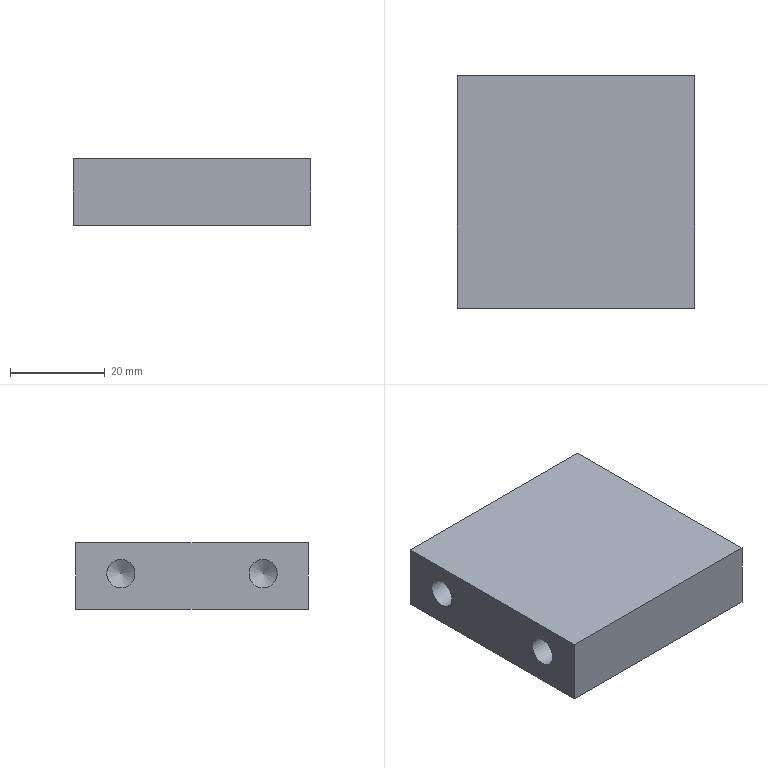Component | NX | BASE_PLATE | 1 solid | 16 faces | box 50 x 49 x 14 mm | volume 32394 mm3 | plane 6 | cone 5 | cylinder 5 | commonest cylinder face diameters 6 x4 4 x1
STEP:
#1=CARTESIAN_POINT('',(0.,0.,0.));
#2=DIRECTION('',(0.,0.,1.));
#3=DIRECTION('',(1.,0.,0.));
#4=AXIS2_PLACEMENT_3D('',#1,#2,#3);
#5=CARTESIAN_POINT('',(25.,0.,2.5));
#6=VERTEX_POINT('',#5);
#7=CARTESIAN_POINT('',(25.,0.,0.5));
#8=DIRECTION('',(-1.,0.,0.));
#9=DIRECTION('',(0.,0.,1.));
#10=AXIS2_PLACEMENT_3D('',#7,#8,#9);
#11=CIRCLE('',#10,2.);
#12=CARTESIAN_POINT('',(25.,-24.5,7.));
#13=DIRECTION('',(-1.,0.,0.));
#14=DIRECTION('',(0.,0.,1.));
#15=AXIS2_PLACEMENT_3D('',#12,#13,#14);
#16=PLANE('',#15);
#17=CARTESIAN_POINT('',(-6.5,24.5));
#18=DIRECTION('',(1.,0.));
#19=AXIS2_PLACEMENT_2D('',#17,#18);
#20=CIRCLE('',#19,2.);
#21=(GEOMETRIC_REPRESENTATION_CONTEXT(2)PARAMETRIC_REPRESENTATION_CONTEXT()REPRESENTATION_CONTEXT('',''));
#22=DEFINITIONAL_REPRESENTATION('',(#20),#21);
#23=PCURVE('',#16,#22);
#24=CARTESIAN_POINT('',(25.,0.,0.5));
#25=DIRECTION('',(-1.,0.,0.));
#26=DIRECTION('',(0.,0.,1.));
#27=AXIS2_PLACEMENT_3D('',#24,#25,#26);
#28=CYLINDRICAL_SURFACE('',#27,2.);
#29=CARTESIAN_POINT('',(0.,0.));
#30=DIRECTION('',(1.,0.));
#31=VECTOR('',#30,1.);
#32=LINE('',#29,#31);
#33=(GEOMETRIC_REPRESENTATION_CONTEXT(2)PARAMETRIC_REPRESENTATION_CONTEXT()REPRESENTATION_CONTEXT('',''));
#34=DEFINITIONAL_REPRESENTATION('',(#32),#33);
#35=PCURVE('',#28,#34);
#36=SURFACE_CURVE('',#11,(#23,#35),.PCURVE_S1.);
#37=EDGE_CURVE('',#6,#6,#36,.T.);
#38=ORIENTED_EDGE('',*,*,#37,.T.);
#39=EDGE_LOOP('',(#38));
#40=FACE_BOUND('',#39,.T.);
#41=CARTESIAN_POINT('',(25.,15.,3.5));
#42=VERTEX_POINT('',#41);
#43=CARTESIAN_POINT('',(25.,15.,0.5));
#44=DIRECTION('',(-1.,0.,0.));
#45=DIRECTION('',(0.,0.,1.));
#46=AXIS2_PLACEMENT_3D('',#43,#44,#45);
#47=CIRCLE('',#46,3.);
#48=CARTESIAN_POINT('',(-6.5,39.5));
#49=DIRECTION('',(1.,0.));
#50=AXIS2_PLACEMENT_2D('',#48,#49);
#51=CIRCLE('',#50,3.);
#52=(GEOMETRIC_REPRESENTATION_CONTEXT(2)PARAMETRIC_REPRESENTATION_CONTEXT()REPRESENTATION_CONTEXT('',''));
#53=DEFINITIONAL_REPRESENTATION('',(#51),#52);
#54=PCURVE('',#16,#53);
#55=CARTESIAN_POINT('',(25.,15.,0.5));
#56=DIRECTION('',(-1.,0.,0.));
#57=DIRECTION('',(0.,0.,1.));
#58=AXIS2_PLACEMENT_3D('',#55,#56,#57);
#59=CYLINDRICAL_SURFACE('',#58,3.);
#60=CARTESIAN_POINT('',(0.,0.));
#61=DIRECTION('',(1.,0.));
#62=VECTOR('',#61,1.);
#63=LINE('',#60,#62);
#64=(GEOMETRIC_REPRESENTATION_CONTEXT(2)PARAMETRIC_REPRESENTATION_CONTEXT()REPRESENTATION_CONTEXT('',''));
#65=DEFINITIONAL_REPRESENTATION('',(#63),#64);
#66=PCURVE('',#59,#65);
#67=SURFACE_CURVE('',#47,(#54,#66),.PCURVE_S1.);
#68=EDGE_CURVE('',#42,#42,#67,.T.);
#69=ORIENTED_EDGE('',*,*,#68,.T.);
#70=EDGE_LOOP('',(#69));
#71=FACE_BOUND('',#70,.T.);
#72=CARTESIAN_POINT('',(25.,-15.,3.5));
#73=VERTEX_POINT('',#72);
#74=CARTESIAN_POINT('',(25.,-15.,0.5));
#75=DIRECTION('',(-1.,0.,0.));
#76=DIRECTION('',(0.,0.,1.));
#77=AXIS2_PLACEMENT_3D('',#74,#75,#76);
#78=CIRCLE('',#77,3.);
#79=CARTESIAN_POINT('',(-6.5,9.5));
#80=DIRECTION('',(1.,0.));
#81=AXIS2_PLACEMENT_2D('',#79,#80);
#82=CIRCLE('',#81,3.);
#83=(GEOMETRIC_REPRESENTATION_CONTEXT(2)PARAMETRIC_REPRESENTATION_CONTEXT()REPRESENTATION_CONTEXT('',''));
#84=DEFINITIONAL_REPRESENTATION('',(#82),#83);
#85=PCURVE('',#16,#84);
#86=CARTESIAN_POINT('',(25.,-15.,0.5));
#87=DIRECTION('',(-1.,0.,0.));
#88=DIRECTION('',(0.,0.,1.));
#89=AXIS2_PLACEMENT_3D('',#86,#87,#88);
#90=CYLINDRICAL_SURFACE('',#89,3.);
#91=CARTESIAN_POINT('',(0.,0.));
#92=DIRECTION('',(1.,0.));
#93=VECTOR('',#92,1.);
#94=LINE('',#91,#93);
#95=(GEOMETRIC_REPRESENTATION_CONTEXT(2)PARAMETRIC_REPRESENTATION_CONTEXT()REPRESENTATION_CONTEXT('',''));
#96=DEFINITIONAL_REPRESENTATION('',(#94),#95);
#97=PCURVE('',#90,#96);
#98=SURFACE_CURVE('',#78,(#85,#97),.PCURVE_S1.);
#99=EDGE_CURVE('',#73,#73,#98,.T.);
#100=ORIENTED_EDGE('',*,*,#99,.T.);
#101=EDGE_LOOP('',(#100));
#102=FACE_BOUND('',#101,.T.);
#103=CARTESIAN_POINT('',(25.,-24.5,-7.));
#104=VERTEX_POINT('',#103);
#105=CARTESIAN_POINT('',(25.,24.5,-7.));
#106=VERTEX_POINT('',#105);
#107=CARTESIAN_POINT('',(25.,-24.5,-7.));
#108=DIRECTION('',(0.,1.,0.));
#109=VECTOR('',#108,1.);
#110=LINE('',#107,#109);
#111=CARTESIAN_POINT('',(-14.,0.));
#112=DIRECTION('',(0.,1.));
#113=VECTOR('',#112,1.);
#114=LINE('',#111,#113);
#115=(GEOMETRIC_REPRESENTATION_CONTEXT(2)PARAMETRIC_REPRESENTATION_CONTEXT()REPRESENTATION_CONTEXT('',''));
#116=DEFINITIONAL_REPRESENTATION('',(#114),#115);
#117=PCURVE('',#16,#116);
#118=CARTESIAN_POINT('',(-25.,-24.5,-7.));
#119=DIRECTION('',(0.,0.,1.));
#120=DIRECTION('',(1.,0.,0.));
#121=AXIS2_PLACEMENT_3D('',#118,#119,#120);
#122=PLANE('',#121);
#123=CARTESIAN_POINT('',(50.,0.));
#124=DIRECTION('',(0.,1.));
#125=VECTOR('',#124,1.);
#126=LINE('',#123,#125);
#127=(GEOMETRIC_REPRESENTATION_CONTEXT(2)PARAMETRIC_REPRESENTATION_CONTEXT()REPRESENTATION_CONTEXT('',''));
#128=DEFINITIONAL_REPRESENTATION('',(#126),#127);
#129=PCURVE('',#122,#128);
#130=SURFACE_CURVE('',#110,(#117,#129),.PCURVE_S1.);
#131=EDGE_CURVE('',#104,#106,#130,.T.);
#132=ORIENTED_EDGE('',*,*,#131,.T.);
#133=CARTESIAN_POINT('',(25.,24.5,7.));
#134=VERTEX_POINT('',#133);
#135=CARTESIAN_POINT('',(25.,24.5,7.));
#136=DIRECTION('',(0.,0.,-1.));
#137=VECTOR('',#136,1.);
#138=LINE('',#135,#137);
#139=CARTESIAN_POINT('',(0.,49.));
#140=DIRECTION('',(-1.,0.));
#141=VECTOR('',#140,1.);
#142=LINE('',#139,#141);
#143=(GEOMETRIC_REPRESENTATION_CONTEXT(2)PARAMETRIC_REPRESENTATION_CONTEXT()REPRESENTATION_CONTEXT('',''));
#144=DEFINITIONAL_REPRESENTATION('',(#142),#143);
#145=PCURVE('',#16,#144);
#146=CARTESIAN_POINT('',(25.,24.5,7.));
#147=DIRECTION('',(0.,-1.,0.));
#148=DIRECTION('',(1.,0.,0.));
#149=AXIS2_PLACEMENT_3D('',#146,#147,#148);
#150=PLANE('',#149);
#151=CARTESIAN_POINT('',(0.,0.));
#152=DIRECTION('',(0.,-1.));
#153=VECTOR('',#152,1.);
#154=LINE('',#151,#153);
#155=(GEOMETRIC_REPRESENTATION_CONTEXT(2)PARAMETRIC_REPRESENTATION_CONTEXT()REPRESENTATION_CONTEXT('',''));
#156=DEFINITIONAL_REPRESENTATION('',(#154),#155);
#157=PCURVE('',#150,#156);
#158=SURFACE_CURVE('',#138,(#145,#157),.PCURVE_S1.);
#159=EDGE_CURVE('',#134,#106,#158,.T.);
#160=ORIENTED_EDGE('',*,*,#159,.F.);
#161=CARTESIAN_POINT('',(25.,-24.5,7.));
#162=VERTEX_POINT('',#161);
#163=CARTESIAN_POINT('',(25.,-24.5,7.));
#164=DIRECTION('',(0.,1.,0.));
#165=VECTOR('',#164,1.);
#166=LINE('',#163,#165);
#167=CARTESIAN_POINT('',(0.,0.));
#168=DIRECTION('',(0.,1.));
#169=VECTOR('',#168,1.);
#170=LINE('',#167,#169);
#171=(GEOMETRIC_REPRESENTATION_CONTEXT(2)PARAMETRIC_REPRESENTATION_CONTEXT()REPRESENTATION_CONTEXT('',''));
#172=DEFINITIONAL_REPRESENTATION('',(#170),#171);
#173=PCURVE('',#16,#172);
#174=CARTESIAN_POINT('',(-25.,-24.5,7.));
#175=DIRECTION('',(0.,0.,1.));
#176=DIRECTION('',(1.,0.,0.));
#177=AXIS2_PLACEMENT_3D('',#174,#175,#176);
#178=PLANE('',#177);
#179=CARTESIAN_POINT('',(50.,0.));
#180=DIRECTION('',(0.,1.));
#181=VECTOR('',#180,1.);
#182=LINE('',#179,#181);
#183=(GEOMETRIC_REPRESENTATION_CONTEXT(2)PARAMETRIC_REPRESENTATION_CONTEXT()REPRESENTATION_CONTEXT('',''));
#184=DEFINITIONAL_REPRESENTATION('',(#182),#183);
#185=PCURVE('',#178,#184);
#186=SURFACE_CURVE('',#166,(#173,#185),.PCURVE_S1.);
#187=EDGE_CURVE('',#162,#134,#186,.T.);
#188=ORIENTED_EDGE('',*,*,#187,.F.);
#189=CARTESIAN_POINT('',(25.,-24.5,7.));
#190=DIRECTION('',(0.,0.,-1.));
#191=VECTOR('',#190,1.);
#192=LINE('',#189,#191);
#193=CARTESIAN_POINT('',(0.,0.));
#194=DIRECTION('',(-1.,0.));
#195=VECTOR('',#194,1.);
#196=LINE('',#193,#195);
#197=(GEOMETRIC_REPRESENTATION_CONTEXT(2)PARAMETRIC_REPRESENTATION_CONTEXT()REPRESENTATION_CONTEXT('',''));
#198=DEFINITIONAL_REPRESENTATION('',(#196),#197);
#199=PCURVE('',#16,#198);
#200=CARTESIAN_POINT('',(-25.,-24.5,7.));
#201=DIRECTION('',(0.,1.,0.));
#202=DIRECTION('',(0.,0.,1.));
#203=AXIS2_PLACEMENT_3D('',#200,#201,#202);
#204=PLANE('',#203);
#205=CARTESIAN_POINT('',(0.,50.));
#206=DIRECTION('',(-1.,0.));
#207=VECTOR('',#206,1.);
#208=LINE('',#205,#207);
#209=(GEOMETRIC_REPRESENTATION_CONTEXT(2)PARAMETRIC_REPRESENTATION_CONTEXT()REPRESENTATION_CONTEXT('',''));
#210=DEFINITIONAL_REPRESENTATION('',(#208),#209);
#211=PCURVE('',#204,#210);
#212=SURFACE_CURVE('',#192,(#199,#211),.PCURVE_S1.);
#213=EDGE_CURVE('',#162,#104,#212,.T.);
#214=ORIENTED_EDGE('',*,*,#213,.T.);
#215=EDGE_LOOP('',(#132,#160,#188,#214));
#216=FACE_BOUND('',#215,.T.);
#217=ADVANCED_FACE('',(#40,#71,#102,#216),#16,.F.);
#218=CARTESIAN_POINT('',(-25.,24.5,-7.));
#219=VERTEX_POINT('',#218);
#220=CARTESIAN_POINT('',(25.,24.5,-7.));
#221=DIRECTION('',(-1.,-0.,0.));
#222=VECTOR('',#221,1.);
#223=LINE('',#220,#222);
#224=CARTESIAN_POINT('',(0.,-14.));
#225=DIRECTION('',(-1.,0.));
#226=VECTOR('',#225,1.);
#227=LINE('',#224,#226);
#228=(GEOMETRIC_REPRESENTATION_CONTEXT(2)PARAMETRIC_REPRESENTATION_CONTEXT()REPRESENTATION_CONTEXT('',''));
#229=DEFINITIONAL_REPRESENTATION('',(#227),#228);
#230=PCURVE('',#150,#229);
#231=CARTESIAN_POINT('',(50.,49.));
#232=DIRECTION('',(-1.,-0.));
#233=VECTOR('',#232,1.);
#234=LINE('',#231,#233);
#235=(GEOMETRIC_REPRESENTATION_CONTEXT(2)PARAMETRIC_REPRESENTATION_CONTEXT()REPRESENTATION_CONTEXT('',''));
#236=DEFINITIONAL_REPRESENTATION('',(#234),#235);
#237=PCURVE('',#122,#236);
#238=SURFACE_CURVE('',#223,(#230,#237),.PCURVE_S1.);
#239=EDGE_CURVE('',#106,#219,#238,.T.);
#240=ORIENTED_EDGE('',*,*,#239,.T.);
#241=CARTESIAN_POINT('',(-25.,24.5,7.));
#242=VERTEX_POINT('',#241);
#243=CARTESIAN_POINT('',(-25.,24.5,7.));
#244=DIRECTION('',(0.,0.,-1.));
#245=VECTOR('',#244,1.);
#246=LINE('',#243,#245);
#247=CARTESIAN_POINT('',(-50.,0.));
#248=DIRECTION('',(0.,-1.));
#249=VECTOR('',#248,1.);
#250=LINE('',#247,#249);
#251=(GEOMETRIC_REPRESENTATION_CONTEXT(2)PARAMETRIC_REPRESENTATION_CONTEXT()REPRESENTATION_CONTEXT('',''));
#252=DEFINITIONAL_REPRESENTATION('',(#250),#251);
#253=PCURVE('',#150,#252);
#254=CARTESIAN_POINT('',(-25.,24.5,7.));
#255=DIRECTION('',(1.,0.,0.));
#256=DIRECTION('',(-0.,1.,0.));
#257=AXIS2_PLACEMENT_3D('',#254,#255,#256);
#258=PLANE('',#257);
#259=CARTESIAN_POINT('',(0.,0.));
#260=DIRECTION('',(0.,-1.));
#261=VECTOR('',#260,1.);
#262=LINE('',#259,#261);
#263=(GEOMETRIC_REPRESENTATION_CONTEXT(2)PARAMETRIC_REPRESENTATION_CONTEXT()REPRESENTATION_CONTEXT('',''));
#264=DEFINITIONAL_REPRESENTATION('',(#262),#263);
#265=PCURVE('',#258,#264);
#266=SURFACE_CURVE('',#246,(#253,#265),.PCURVE_S1.);
#267=EDGE_CURVE('',#242,#219,#266,.T.);
#268=ORIENTED_EDGE('',*,*,#267,.F.);
#269=CARTESIAN_POINT('',(25.,24.5,7.));
#270=DIRECTION('',(-1.,-0.,0.));
#271=VECTOR('',#270,1.);
#272=LINE('',#269,#271);
#273=CARTESIAN_POINT('',(0.,0.));
#274=DIRECTION('',(-1.,0.));
#275=VECTOR('',#274,1.);
#276=LINE('',#273,#275);
#277=(GEOMETRIC_REPRESENTATION_CONTEXT(2)PARAMETRIC_REPRESENTATION_CONTEXT()REPRESENTATION_CONTEXT('',''));
#278=DEFINITIONAL_REPRESENTATION('',(#276),#277);
#279=PCURVE('',#150,#278);
#280=CARTESIAN_POINT('',(50.,49.));
#281=DIRECTION('',(-1.,-0.));
#282=VECTOR('',#281,1.);
#283=LINE('',#280,#282);
#284=(GEOMETRIC_REPRESENTATION_CONTEXT(2)PARAMETRIC_REPRESENTATION_CONTEXT()REPRESENTATION_CONTEXT('',''));
#285=DEFINITIONAL_REPRESENTATION('',(#283),#284);
#286=PCURVE('',#178,#285);
#287=SURFACE_CURVE('',#272,(#279,#286),.PCURVE_S1.);
#288=EDGE_CURVE('',#134,#242,#287,.T.);
#289=ORIENTED_EDGE('',*,*,#288,.F.);
#290=ORIENTED_EDGE('',*,*,#159,.T.);
#291=EDGE_LOOP('',(#240,#268,#289,#290));
#292=FACE_BOUND('',#291,.T.);
#293=ADVANCED_FACE('',(#292),#150,.F.);
#294=CARTESIAN_POINT('',(-25.,15.,-2.5));
#295=VERTEX_POINT('',#294);
#296=CARTESIAN_POINT('',(-25.,15.,0.5));
#297=DIRECTION('',(1.,0.,0.));
#298=DIRECTION('',(0.,0.,-1.));
#299=AXIS2_PLACEMENT_3D('',#296,#297,#298);
#300=CIRCLE('',#299,3.);
#301=CARTESIAN_POINT('',(-9.5,-6.5));
#302=DIRECTION('',(0.,-1.));
#303=AXIS2_PLACEMENT_2D('',#301,#302);
#304=CIRCLE('',#303,3.);
#305=(GEOMETRIC_REPRESENTATION_CONTEXT(2)PARAMETRIC_REPRESENTATION_CONTEXT()REPRESENTATION_CONTEXT('',''));
#306=DEFINITIONAL_REPRESENTATION('',(#304),#305);
#307=PCURVE('',#258,#306);
#308=CARTESIAN_POINT('',(-25.,15.,0.5));
#309=DIRECTION('',(1.,0.,0.));
#310=DIRECTION('',(0.,0.,-1.));
#311=AXIS2_PLACEMENT_3D('',#308,#309,#310);
#312=CYLINDRICAL_SURFACE('',#311,3.);
#313=CARTESIAN_POINT('',(0.,0.));
#314=DIRECTION('',(1.,0.));
#315=VECTOR('',#314,1.);
#316=LINE('',#313,#315);
#317=(GEOMETRIC_REPRESENTATION_CONTEXT(2)PARAMETRIC_REPRESENTATION_CONTEXT()REPRESENTATION_CONTEXT('',''));
#318=DEFINITIONAL_REPRESENTATION('',(#316),#317);
#319=PCURVE('',#312,#318);
#320=SURFACE_CURVE('',#300,(#307,#319),.PCURVE_S1.);
#321=EDGE_CURVE('',#295,#295,#320,.T.);
#322=ORIENTED_EDGE('',*,*,#321,.T.);
#323=EDGE_LOOP('',(#322));
#324=FACE_BOUND('',#323,.T.);
#325=CARTESIAN_POINT('',(-25.,-15.,-2.5));
#326=VERTEX_POINT('',#325);
#327=CARTESIAN_POINT('',(-25.,-15.,0.5));
#328=DIRECTION('',(1.,0.,0.));
#329=DIRECTION('',(0.,0.,-1.));
#330=AXIS2_PLACEMENT_3D('',#327,#328,#329);
#331=CIRCLE('',#330,3.);
#332=CARTESIAN_POINT('',(-39.5,-6.5));
#333=DIRECTION('',(0.,-1.));
#334=AXIS2_PLACEMENT_2D('',#332,#333);
#335=CIRCLE('',#334,3.);
#336=(GEOMETRIC_REPRESENTATION_CONTEXT(2)PARAMETRIC_REPRESENTATION_CONTEXT()REPRESENTATION_CONTEXT('',''));
#337=DEFINITIONAL_REPRESENTATION('',(#335),#336);
#338=PCURVE('',#258,#337);
#339=CARTESIAN_POINT('',(-25.,-15.,0.5));
#340=DIRECTION('',(1.,0.,0.));
#341=DIRECTION('',(0.,0.,-1.));
#342=AXIS2_PLACEMENT_3D('',#339,#340,#341);
#343=CYLINDRICAL_SURFACE('',#342,3.);
#344=CARTESIAN_POINT('',(0.,0.));
#345=DIRECTION('',(1.,0.));
#346=VECTOR('',#345,1.);
#347=LINE('',#344,#346);
#348=(GEOMETRIC_REPRESENTATION_CONTEXT(2)PARAMETRIC_REPRESENTATION_CONTEXT()REPRESENTATION_CONTEXT('',''));
#349=DEFINITIONAL_REPRESENTATION('',(#347),#348);
#350=PCURVE('',#343,#349);
#351=SURFACE_CURVE('',#331,(#338,#350),.PCURVE_S1.);
#352=EDGE_CURVE('',#326,#326,#351,.T.);
#353=ORIENTED_EDGE('',*,*,#352,.T.);
#354=EDGE_LOOP('',(#353));
#355=FACE_BOUND('',#354,.T.);
#356=CARTESIAN_POINT('',(-25.,-24.5,-7.));
#357=VERTEX_POINT('',#356);
#358=CARTESIAN_POINT('',(-25.,24.5,-7.));
#359=DIRECTION('',(0.,-1.,0.));
#360=VECTOR('',#359,1.);
#361=LINE('',#358,#360);
#362=CARTESIAN_POINT('',(0.,-14.));
#363=DIRECTION('',(-1.,0.));
#364=VECTOR('',#363,1.);
#365=LINE('',#362,#364);
#366=(GEOMETRIC_REPRESENTATION_CONTEXT(2)PARAMETRIC_REPRESENTATION_CONTEXT()REPRESENTATION_CONTEXT('',''));
#367=DEFINITIONAL_REPRESENTATION('',(#365),#366);
#368=PCURVE('',#258,#367);
#369=CARTESIAN_POINT('',(0.,49.));
#370=DIRECTION('',(0.,-1.));
#371=VECTOR('',#370,1.);
#372=LINE('',#369,#371);
#373=(GEOMETRIC_REPRESENTATION_CONTEXT(2)PARAMETRIC_REPRESENTATION_CONTEXT()REPRESENTATION_CONTEXT('',''));
#374=DEFINITIONAL_REPRESENTATION('',(#372),#373);
#375=PCURVE('',#122,#374);
#376=SURFACE_CURVE('',#361,(#368,#375),.PCURVE_S1.);
#377=EDGE_CURVE('',#219,#357,#376,.T.);
#378=ORIENTED_EDGE('',*,*,#377,.T.);
#379=CARTESIAN_POINT('',(-25.,-24.5,7.));
#380=VERTEX_POINT('',#379);
#381=CARTESIAN_POINT('',(-25.,-24.5,7.));
#382=DIRECTION('',(0.,0.,-1.));
#383=VECTOR('',#382,1.);
#384=LINE('',#381,#383);
#385=CARTESIAN_POINT('',(-49.,0.));
#386=DIRECTION('',(0.,-1.));
#387=VECTOR('',#386,1.);
#388=LINE('',#385,#387);
#389=(GEOMETRIC_REPRESENTATION_CONTEXT(2)PARAMETRIC_REPRESENTATION_CONTEXT()REPRESENTATION_CONTEXT('',''));
#390=DEFINITIONAL_REPRESENTATION('',(#388),#389);
#391=PCURVE('',#258,#390);
#392=CARTESIAN_POINT('',(0.,0.));
#393=DIRECTION('',(-1.,0.));
#394=VECTOR('',#393,1.);
#395=LINE('',#392,#394);
#396=(GEOMETRIC_REPRESENTATION_CONTEXT(2)PARAMETRIC_REPRESENTATION_CONTEXT()REPRESENTATION_CONTEXT('',''));
#397=DEFINITIONAL_REPRESENTATION('',(#395),#396);
#398=PCURVE('',#204,#397);
#399=SURFACE_CURVE('',#384,(#391,#398),.PCURVE_S1.);
#400=EDGE_CURVE('',#380,#357,#399,.T.);
#401=ORIENTED_EDGE('',*,*,#400,.F.);
#402=CARTESIAN_POINT('',(-25.,24.5,7.));
#403=DIRECTION('',(0.,-1.,0.));
#404=VECTOR('',#403,1.);
#405=LINE('',#402,#404);
#406=CARTESIAN_POINT('',(0.,0.));
#407=DIRECTION('',(-1.,0.));
#408=VECTOR('',#407,1.);
#409=LINE('',#406,#408);
#410=(GEOMETRIC_REPRESENTATION_CONTEXT(2)PARAMETRIC_REPRESENTATION_CONTEXT()REPRESENTATION_CONTEXT('',''));
#411=DEFINITIONAL_REPRESENTATION('',(#409),#410);
#412=PCURVE('',#258,#411);
#413=CARTESIAN_POINT('',(0.,49.));
#414=DIRECTION('',(0.,-1.));
#415=VECTOR('',#414,1.);
#416=LINE('',#413,#415);
#417=(GEOMETRIC_REPRESENTATION_CONTEXT(2)PARAMETRIC_REPRESENTATION_CONTEXT()REPRESENTATION_CONTEXT('',''));
#418=DEFINITIONAL_REPRESENTATION('',(#416),#417);
#419=PCURVE('',#178,#418);
#420=SURFACE_CURVE('',#405,(#412,#419),.PCURVE_S1.);
#421=EDGE_CURVE('',#242,#380,#420,.T.);
#422=ORIENTED_EDGE('',*,*,#421,.F.);
#423=ORIENTED_EDGE('',*,*,#267,.T.);
#424=EDGE_LOOP('',(#378,#401,#422,#423));
#425=FACE_BOUND('',#424,.T.);
#426=ADVANCED_FACE('',(#324,#355,#425),#258,.F.);
#427=CARTESIAN_POINT('',(-25.,-24.5,-7.));
#428=DIRECTION('',(1.,0.,0.));
#429=VECTOR('',#428,1.);
#430=LINE('',#427,#429);
#431=CARTESIAN_POINT('',(-14.,0.));
#432=DIRECTION('',(0.,1.));
#433=VECTOR('',#432,1.);
#434=LINE('',#431,#433);
#435=(GEOMETRIC_REPRESENTATION_CONTEXT(2)PARAMETRIC_REPRESENTATION_CONTEXT()REPRESENTATION_CONTEXT('',''));
#436=DEFINITIONAL_REPRESENTATION('',(#434),#435);
#437=PCURVE('',#204,#436);
#438=CARTESIAN_POINT('',(0.,0.));
#439=DIRECTION('',(1.,0.));
#440=VECTOR('',#439,1.);
#441=LINE('',#438,#440);
#442=(GEOMETRIC_REPRESENTATION_CONTEXT(2)PARAMETRIC_REPRESENTATION_CONTEXT()REPRESENTATION_CONTEXT('',''));
#443=DEFINITIONAL_REPRESENTATION('',(#441),#442);
#444=PCURVE('',#122,#443);
#445=SURFACE_CURVE('',#430,(#437,#444),.PCURVE_S1.);
#446=EDGE_CURVE('',#357,#104,#445,.T.);
#447=ORIENTED_EDGE('',*,*,#446,.T.);
#448=ORIENTED_EDGE('',*,*,#213,.F.);
#449=CARTESIAN_POINT('',(-25.,-24.5,7.));
#450=DIRECTION('',(1.,0.,0.));
#451=VECTOR('',#450,1.);
#452=LINE('',#449,#451);
#453=CARTESIAN_POINT('',(0.,0.));
#454=DIRECTION('',(0.,1.));
#455=VECTOR('',#454,1.);
#456=LINE('',#453,#455);
#457=(GEOMETRIC_REPRESENTATION_CONTEXT(2)PARAMETRIC_REPRESENTATION_CONTEXT()REPRESENTATION_CONTEXT('',''));
#458=DEFINITIONAL_REPRESENTATION('',(#456),#457);
#459=PCURVE('',#204,#458);
#460=CARTESIAN_POINT('',(0.,0.));
#461=DIRECTION('',(1.,0.));
#462=VECTOR('',#461,1.);
#463=LINE('',#460,#462);
#464=(GEOMETRIC_REPRESENTATION_CONTEXT(2)PARAMETRIC_REPRESENTATION_CONTEXT()REPRESENTATION_CONTEXT('',''));
#465=DEFINITIONAL_REPRESENTATION('',(#463),#464);
#466=PCURVE('',#178,#465);
#467=SURFACE_CURVE('',#452,(#459,#466),.PCURVE_S1.);
#468=EDGE_CURVE('',#380,#162,#467,.T.);
#469=ORIENTED_EDGE('',*,*,#468,.F.);
#470=ORIENTED_EDGE('',*,*,#400,.T.);
#471=EDGE_LOOP('',(#447,#448,#469,#470));
#472=FACE_BOUND('',#471,.T.);
#473=ADVANCED_FACE('',(#472),#204,.F.);
#474=ORIENTED_EDGE('',*,*,#187,.T.);
#475=ORIENTED_EDGE('',*,*,#288,.T.);
#476=ORIENTED_EDGE('',*,*,#421,.T.);
#477=ORIENTED_EDGE('',*,*,#468,.T.);
#478=EDGE_LOOP('',(#474,#475,#476,#477));
#479=FACE_BOUND('',#478,.T.);
#480=ADVANCED_FACE('',(#479),#178,.T.);
#481=ORIENTED_EDGE('',*,*,#131,.F.);
#482=ORIENTED_EDGE('',*,*,#446,.F.);
#483=ORIENTED_EDGE('',*,*,#377,.F.);
#484=ORIENTED_EDGE('',*,*,#239,.F.);
#485=EDGE_LOOP('',(#481,#482,#483,#484));
#486=FACE_BOUND('',#485,.T.);
#487=ADVANCED_FACE('',(#486),#122,.F.);
#488=CARTESIAN_POINT('',(9.9,-15.,-2.5));
#489=VERTEX_POINT('',#488);
#490=CARTESIAN_POINT('',(9.9,-15.,3.5));
#491=VERTEX_POINT('',#490);
#492=CARTESIAN_POINT('',(9.9,-15.,0.5));
#493=DIRECTION('',(1.,0.,0.));
#494=DIRECTION('',(0.,0.,1.));
#495=AXIS2_PLACEMENT_3D('',#492,#493,#494);
#496=CIRCLE('',#495,3.);
#497=CARTESIAN_POINT('',(9.9,-15.,0.5));
#498=DIRECTION('',(1.,0.,0.));
#499=DIRECTION('',(0.,0.,-1.));
#500=AXIS2_PLACEMENT_3D('',#497,#498,#499);
#501=CONICAL_SURFACE('',#500,3.,1.03);
#502=CARTESIAN_POINT('',(-3.142,0.));
#503=DIRECTION('',(1.,0.));
#504=VECTOR('',#503,1.);
#505=LINE('',#502,#504);
#506=(GEOMETRIC_REPRESENTATION_CONTEXT(2)PARAMETRIC_REPRESENTATION_CONTEXT()REPRESENTATION_CONTEXT('',''));
#507=DEFINITIONAL_REPRESENTATION('',(#505),#506);
#508=PCURVE('',#501,#507);
#509=CARTESIAN_POINT('',(6.283,15.1));
#510=DIRECTION('',(-1.,0.));
#511=VECTOR('',#510,1.);
#512=LINE('',#509,#511);
#513=(GEOMETRIC_REPRESENTATION_CONTEXT(2)PARAMETRIC_REPRESENTATION_CONTEXT()REPRESENTATION_CONTEXT('',''));
#514=DEFINITIONAL_REPRESENTATION('',(#512),#513);
#515=PCURVE('',#90,#514);
#516=SURFACE_CURVE('',#496,(#508,#515),.PCURVE_S1.);
#517=EDGE_CURVE('',#489,#491,#516,.T.);
#518=ORIENTED_EDGE('',*,*,#517,.F.);
#519=CARTESIAN_POINT('',(8.097,-15.,0.5));
#520=VERTEX_POINT('',#519);
#521=CARTESIAN_POINT('',(8.097,-15.,0.5));
#522=CARTESIAN_POINT('',(9.9,-15.,-2.5));
#523=B_SPLINE_CURVE_WITH_KNOTS('',1,(#521,#522),.UNSPECIFIED.,.F.,.F.,(2,2),(-3.5,0.),.PIECEWISE_BEZIER_KNOTS.);
#524=CARTESIAN_POINT('',(0.,0.));
#525=DIRECTION('',(0.,1.));
#526=VECTOR('',#525,1.);
#527=LINE('',#524,#526);
#528=(GEOMETRIC_REPRESENTATION_CONTEXT(2)PARAMETRIC_REPRESENTATION_CONTEXT()REPRESENTATION_CONTEXT('',''));
#529=DEFINITIONAL_REPRESENTATION('',(#527),#528);
#530=PCURVE('',#501,#529);
#531=CARTESIAN_POINT('',(6.283,0.));
#532=DIRECTION('',(0.,1.));
#533=VECTOR('',#532,1.);
#534=LINE('',#531,#533);
#535=(GEOMETRIC_REPRESENTATION_CONTEXT(2)PARAMETRIC_REPRESENTATION_CONTEXT()REPRESENTATION_CONTEXT('',''));
#536=DEFINITIONAL_REPRESENTATION('',(#534),#535);
#537=PCURVE('',#501,#536);
#538=SEAM_CURVE('',#523,(#530,#537),.PCURVE_S1.);
#539=EDGE_CURVE('',#520,#489,#538,.T.);
#540=ORIENTED_EDGE('',*,*,#539,.F.);
#541=ORIENTED_EDGE('',*,*,#539,.T.);
#542=CARTESIAN_POINT('',(9.9,-15.,0.5));
#543=DIRECTION('',(1.,0.,0.));
#544=DIRECTION('',(0.,0.,1.));
#545=AXIS2_PLACEMENT_3D('',#542,#543,#544);
#546=CIRCLE('',#545,3.);
#547=CARTESIAN_POINT('',(3.142,0.));
#548=DIRECTION('',(1.,0.));
#549=VECTOR('',#548,1.);
#550=LINE('',#547,#549);
#551=(GEOMETRIC_REPRESENTATION_CONTEXT(2)PARAMETRIC_REPRESENTATION_CONTEXT()REPRESENTATION_CONTEXT('',''));
#552=DEFINITIONAL_REPRESENTATION('',(#550),#551);
#553=PCURVE('',#501,#552);
#554=CARTESIAN_POINT('',(6.283,15.1));
#555=DIRECTION('',(-1.,0.));
#556=VECTOR('',#555,1.);
#557=LINE('',#554,#556);
#558=(GEOMETRIC_REPRESENTATION_CONTEXT(2)PARAMETRIC_REPRESENTATION_CONTEXT()REPRESENTATION_CONTEXT('',''));
#559=DEFINITIONAL_REPRESENTATION('',(#557),#558);
#560=PCURVE('',#90,#559);
#561=SURFACE_CURVE('',#546,(#553,#560),.PCURVE_S1.);
#562=EDGE_CURVE('',#491,#489,#561,.T.);
#563=ORIENTED_EDGE('',*,*,#562,.F.);
#564=EDGE_LOOP('',(#518,#540,#541,#563));
#565=FACE_BOUND('',#564,.F.);
#566=ADVANCED_FACE('',(#565),#501,.F.);
#567=ORIENTED_EDGE('',*,*,#517,.T.);
#568=CARTESIAN_POINT('',(25.,-15.,3.5));
#569=CARTESIAN_POINT('',(9.9,-15.,3.5));
#570=B_SPLINE_CURVE_WITH_KNOTS('',1,(#568,#569),.UNSPECIFIED.,.F.,.F.,(2,2),(0.,15.1),.PIECEWISE_BEZIER_KNOTS.);
#571=CARTESIAN_POINT('',(0.,0.));
#572=DIRECTION('',(0.,1.));
#573=VECTOR('',#572,1.);
#574=LINE('',#571,#573);
#575=(GEOMETRIC_REPRESENTATION_CONTEXT(2)PARAMETRIC_REPRESENTATION_CONTEXT()REPRESENTATION_CONTEXT('',''));
#576=DEFINITIONAL_REPRESENTATION('',(#574),#575);
#577=PCURVE('',#90,#576);
#578=CARTESIAN_POINT('',(6.283,0.));
#579=DIRECTION('',(0.,1.));
#580=VECTOR('',#579,1.);
#581=LINE('',#578,#580);
#582=(GEOMETRIC_REPRESENTATION_CONTEXT(2)PARAMETRIC_REPRESENTATION_CONTEXT()REPRESENTATION_CONTEXT('',''));
#583=DEFINITIONAL_REPRESENTATION('',(#581),#582);
#584=PCURVE('',#90,#583);
#585=SEAM_CURVE('',#570,(#577,#584),.PCURVE_S1.);
#586=EDGE_CURVE('',#73,#491,#585,.T.);
#587=ORIENTED_EDGE('',*,*,#586,.F.);
#588=ORIENTED_EDGE('',*,*,#99,.T.);
#589=ORIENTED_EDGE('',*,*,#586,.T.);
#590=ORIENTED_EDGE('',*,*,#562,.T.);
#591=EDGE_LOOP('',(#567,#587,#588,#589,#590));
#592=FACE_BOUND('',#591,.F.);
#593=ADVANCED_FACE('',(#592),#90,.F.);
#594=CARTESIAN_POINT('',(9.9,15.,-2.5));
#595=VERTEX_POINT('',#594);
#596=CARTESIAN_POINT('',(9.9,15.,3.5));
#597=VERTEX_POINT('',#596);
#598=CARTESIAN_POINT('',(9.9,15.,0.5));
#599=DIRECTION('',(1.,0.,0.));
#600=DIRECTION('',(0.,0.,1.));
#601=AXIS2_PLACEMENT_3D('',#598,#599,#600);
#602=CIRCLE('',#601,3.);
#603=CARTESIAN_POINT('',(9.9,15.,0.5));
#604=DIRECTION('',(1.,0.,0.));
#605=DIRECTION('',(0.,0.,-1.));
#606=AXIS2_PLACEMENT_3D('',#603,#604,#605);
#607=CONICAL_SURFACE('',#606,3.,1.03);
#608=CARTESIAN_POINT('',(-3.142,0.));
#609=DIRECTION('',(1.,0.));
#610=VECTOR('',#609,1.);
#611=LINE('',#608,#610);
#612=(GEOMETRIC_REPRESENTATION_CONTEXT(2)PARAMETRIC_REPRESENTATION_CONTEXT()REPRESENTATION_CONTEXT('',''));
#613=DEFINITIONAL_REPRESENTATION('',(#611),#612);
#614=PCURVE('',#607,#613);
#615=CARTESIAN_POINT('',(6.283,15.1));
#616=DIRECTION('',(-1.,0.));
#617=VECTOR('',#616,1.);
#618=LINE('',#615,#617);
#619=(GEOMETRIC_REPRESENTATION_CONTEXT(2)PARAMETRIC_REPRESENTATION_CONTEXT()REPRESENTATION_CONTEXT('',''));
#620=DEFINITIONAL_REPRESENTATION('',(#618),#619);
#621=PCURVE('',#59,#620);
#622=SURFACE_CURVE('',#602,(#614,#621),.PCURVE_S1.);
#623=EDGE_CURVE('',#595,#597,#622,.T.);
#624=ORIENTED_EDGE('',*,*,#623,.F.);
#625=CARTESIAN_POINT('',(8.097,15.,0.5));
#626=VERTEX_POINT('',#625);
#627=CARTESIAN_POINT('',(8.097,15.,0.5));
#628=CARTESIAN_POINT('',(9.9,15.,-2.5));
#629=B_SPLINE_CURVE_WITH_KNOTS('',1,(#627,#628),.UNSPECIFIED.,.F.,.F.,(2,2),(-3.5,0.),.PIECEWISE_BEZIER_KNOTS.);
#630=CARTESIAN_POINT('',(0.,0.));
#631=DIRECTION('',(0.,1.));
#632=VECTOR('',#631,1.);
#633=LINE('',#630,#632);
#634=(GEOMETRIC_REPRESENTATION_CONTEXT(2)PARAMETRIC_REPRESENTATION_CONTEXT()REPRESENTATION_CONTEXT('',''));
#635=DEFINITIONAL_REPRESENTATION('',(#633),#634);
#636=PCURVE('',#607,#635);
#637=CARTESIAN_POINT('',(6.283,0.));
#638=DIRECTION('',(0.,1.));
#639=VECTOR('',#638,1.);
#640=LINE('',#637,#639);
#641=(GEOMETRIC_REPRESENTATION_CONTEXT(2)PARAMETRIC_REPRESENTATION_CONTEXT()REPRESENTATION_CONTEXT('',''));
#642=DEFINITIONAL_REPRESENTATION('',(#640),#641);
#643=PCURVE('',#607,#642);
#644=SEAM_CURVE('',#629,(#636,#643),.PCURVE_S1.);
#645=EDGE_CURVE('',#626,#595,#644,.T.);
#646=ORIENTED_EDGE('',*,*,#645,.F.);
#647=ORIENTED_EDGE('',*,*,#645,.T.);
#648=CARTESIAN_POINT('',(9.9,15.,0.5));
#649=DIRECTION('',(1.,0.,0.));
#650=DIRECTION('',(0.,0.,1.));
#651=AXIS2_PLACEMENT_3D('',#648,#649,#650);
#652=CIRCLE('',#651,3.);
#653=CARTESIAN_POINT('',(3.142,0.));
#654=DIRECTION('',(1.,0.));
#655=VECTOR('',#654,1.);
#656=LINE('',#653,#655);
#657=(GEOMETRIC_REPRESENTATION_CONTEXT(2)PARAMETRIC_REPRESENTATION_CONTEXT()REPRESENTATION_CONTEXT('',''));
#658=DEFINITIONAL_REPRESENTATION('',(#656),#657);
#659=PCURVE('',#607,#658);
#660=CARTESIAN_POINT('',(6.283,15.1));
#661=DIRECTION('',(-1.,0.));
#662=VECTOR('',#661,1.);
#663=LINE('',#660,#662);
#664=(GEOMETRIC_REPRESENTATION_CONTEXT(2)PARAMETRIC_REPRESENTATION_CONTEXT()REPRESENTATION_CONTEXT('',''));
#665=DEFINITIONAL_REPRESENTATION('',(#663),#664);
#666=PCURVE('',#59,#665);
#667=SURFACE_CURVE('',#652,(#659,#666),.PCURVE_S1.);
#668=EDGE_CURVE('',#597,#595,#667,.T.);
#669=ORIENTED_EDGE('',*,*,#668,.F.);
#670=EDGE_LOOP('',(#624,#646,#647,#669));
#671=FACE_BOUND('',#670,.F.);
#672=ADVANCED_FACE('',(#671),#607,.F.);
#673=ORIENTED_EDGE('',*,*,#623,.T.);
#674=CARTESIAN_POINT('',(25.,15.,3.5));
#675=CARTESIAN_POINT('',(9.9,15.,3.5));
#676=B_SPLINE_CURVE_WITH_KNOTS('',1,(#674,#675),.UNSPECIFIED.,.F.,.F.,(2,2),(0.,15.1),.PIECEWISE_BEZIER_KNOTS.);
#677=CARTESIAN_POINT('',(0.,0.));
#678=DIRECTION('',(0.,1.));
#679=VECTOR('',#678,1.);
#680=LINE('',#677,#679);
#681=(GEOMETRIC_REPRESENTATION_CONTEXT(2)PARAMETRIC_REPRESENTATION_CONTEXT()REPRESENTATION_CONTEXT('',''));
#682=DEFINITIONAL_REPRESENTATION('',(#680),#681);
#683=PCURVE('',#59,#682);
#684=CARTESIAN_POINT('',(6.283,0.));
#685=DIRECTION('',(0.,1.));
#686=VECTOR('',#685,1.);
#687=LINE('',#684,#686);
#688=(GEOMETRIC_REPRESENTATION_CONTEXT(2)PARAMETRIC_REPRESENTATION_CONTEXT()REPRESENTATION_CONTEXT('',''));
#689=DEFINITIONAL_REPRESENTATION('',(#687),#688);
#690=PCURVE('',#59,#689);
#691=SEAM_CURVE('',#676,(#683,#690),.PCURVE_S1.);
#692=EDGE_CURVE('',#42,#597,#691,.T.);
#693=ORIENTED_EDGE('',*,*,#692,.F.);
#694=ORIENTED_EDGE('',*,*,#68,.T.);
#695=ORIENTED_EDGE('',*,*,#692,.T.);
#696=ORIENTED_EDGE('',*,*,#668,.T.);
#697=EDGE_LOOP('',(#673,#693,#694,#695,#696));
#698=FACE_BOUND('',#697,.F.);
#699=ADVANCED_FACE('',(#698),#59,.F.);
#700=CARTESIAN_POINT('',(-9.9,-15.,-2.5));
#701=VERTEX_POINT('',#700);
#702=CARTESIAN_POINT('',(-9.9,-15.,3.5));
#703=VERTEX_POINT('',#702);
#704=CARTESIAN_POINT('',(-9.9,-15.,0.5));
#705=DIRECTION('',(1.,0.,0.));
#706=DIRECTION('',(0.,0.,-1.));
#707=AXIS2_PLACEMENT_3D('',#704,#705,#706);
#708=CIRCLE('',#707,3.);
#709=CARTESIAN_POINT('',(-9.9,-15.,0.5));
#710=DIRECTION('',(-1.,0.,0.));
#711=DIRECTION('',(0.,0.,1.));
#712=AXIS2_PLACEMENT_3D('',#709,#710,#711);
#713=CONICAL_SURFACE('',#712,3.,1.03);
#714=CARTESIAN_POINT('',(3.142,0.));
#715=DIRECTION('',(-1.,0.));
#716=VECTOR('',#715,1.);
#717=LINE('',#714,#716);
#718=(GEOMETRIC_REPRESENTATION_CONTEXT(2)PARAMETRIC_REPRESENTATION_CONTEXT()REPRESENTATION_CONTEXT('',''));
#719=DEFINITIONAL_REPRESENTATION('',(#717),#718);
#720=PCURVE('',#713,#719);
#721=CARTESIAN_POINT('',(0.,15.1));
#722=DIRECTION('',(1.,0.));
#723=VECTOR('',#722,1.);
#724=LINE('',#721,#723);
#725=(GEOMETRIC_REPRESENTATION_CONTEXT(2)PARAMETRIC_REPRESENTATION_CONTEXT()REPRESENTATION_CONTEXT('',''));
#726=DEFINITIONAL_REPRESENTATION('',(#724),#725);
#727=PCURVE('',#343,#726);
#728=SURFACE_CURVE('',#708,(#720,#727),.PCURVE_S1.);
#729=EDGE_CURVE('',#701,#703,#728,.T.);
#730=ORIENTED_EDGE('',*,*,#729,.T.);
#731=CARTESIAN_POINT('',(-8.097,-15.,0.5));
#732=VERTEX_POINT('',#731);
#733=CARTESIAN_POINT('',(-8.097,-15.,0.5));
#734=CARTESIAN_POINT('',(-9.9,-15.,3.5));
#735=B_SPLINE_CURVE_WITH_KNOTS('',1,(#733,#734),.UNSPECIFIED.,.F.,.F.,(2,2),(-3.5,0.),.PIECEWISE_BEZIER_KNOTS.);
#736=CARTESIAN_POINT('',(0.,0.));
#737=DIRECTION('',(0.,1.));
#738=VECTOR('',#737,1.);
#739=LINE('',#736,#738);
#740=(GEOMETRIC_REPRESENTATION_CONTEXT(2)PARAMETRIC_REPRESENTATION_CONTEXT()REPRESENTATION_CONTEXT('',''));
#741=DEFINITIONAL_REPRESENTATION('',(#739),#740);
#742=PCURVE('',#713,#741);
#743=CARTESIAN_POINT('',(6.283,0.));
#744=DIRECTION('',(0.,1.));
#745=VECTOR('',#744,1.);
#746=LINE('',#743,#745);
#747=(GEOMETRIC_REPRESENTATION_CONTEXT(2)PARAMETRIC_REPRESENTATION_CONTEXT()REPRESENTATION_CONTEXT('',''));
#748=DEFINITIONAL_REPRESENTATION('',(#746),#747);
#749=PCURVE('',#713,#748);
#750=SEAM_CURVE('',#735,(#742,#749),.PCURVE_S1.);
#751=EDGE_CURVE('',#732,#703,#750,.T.);
#752=ORIENTED_EDGE('',*,*,#751,.F.);
#753=ORIENTED_EDGE('',*,*,#751,.T.);
#754=CARTESIAN_POINT('',(-9.9,-15.,0.5));
#755=DIRECTION('',(1.,0.,0.));
#756=DIRECTION('',(0.,0.,-1.));
#757=AXIS2_PLACEMENT_3D('',#754,#755,#756);
#758=CIRCLE('',#757,3.);
#759=CARTESIAN_POINT('',(9.425,0.));
#760=DIRECTION('',(-1.,0.));
#761=VECTOR('',#760,1.);
#762=LINE('',#759,#761);
#763=(GEOMETRIC_REPRESENTATION_CONTEXT(2)PARAMETRIC_REPRESENTATION_CONTEXT()REPRESENTATION_CONTEXT('',''));
#764=DEFINITIONAL_REPRESENTATION('',(#762),#763);
#765=PCURVE('',#713,#764);
#766=CARTESIAN_POINT('',(0.,15.1));
#767=DIRECTION('',(1.,0.));
#768=VECTOR('',#767,1.);
#769=LINE('',#766,#768);
#770=(GEOMETRIC_REPRESENTATION_CONTEXT(2)PARAMETRIC_REPRESENTATION_CONTEXT()REPRESENTATION_CONTEXT('',''));
#771=DEFINITIONAL_REPRESENTATION('',(#769),#770);
#772=PCURVE('',#343,#771);
#773=SURFACE_CURVE('',#758,(#765,#772),.PCURVE_S1.);
#774=EDGE_CURVE('',#703,#701,#773,.T.);
#775=ORIENTED_EDGE('',*,*,#774,.T.);
#776=EDGE_LOOP('',(#730,#752,#753,#775));
#777=FACE_BOUND('',#776,.F.);
#778=ADVANCED_FACE('',(#777),#713,.F.);
#779=ORIENTED_EDGE('',*,*,#774,.F.);
#780=ORIENTED_EDGE('',*,*,#729,.F.);
#781=CARTESIAN_POINT('',(-25.,-15.,-2.5));
#782=CARTESIAN_POINT('',(-9.9,-15.,-2.5));
#783=B_SPLINE_CURVE_WITH_KNOTS('',1,(#781,#782),.UNSPECIFIED.,.F.,.F.,(2,2),(0.,15.1),.PIECEWISE_BEZIER_KNOTS.);
#784=CARTESIAN_POINT('',(0.,0.));
#785=DIRECTION('',(0.,1.));
#786=VECTOR('',#785,1.);
#787=LINE('',#784,#786);
#788=(GEOMETRIC_REPRESENTATION_CONTEXT(2)PARAMETRIC_REPRESENTATION_CONTEXT()REPRESENTATION_CONTEXT('',''));
#789=DEFINITIONAL_REPRESENTATION('',(#787),#788);
#790=PCURVE('',#343,#789);
#791=CARTESIAN_POINT('',(6.283,0.));
#792=DIRECTION('',(0.,1.));
#793=VECTOR('',#792,1.);
#794=LINE('',#791,#793);
#795=(GEOMETRIC_REPRESENTATION_CONTEXT(2)PARAMETRIC_REPRESENTATION_CONTEXT()REPRESENTATION_CONTEXT('',''));
#796=DEFINITIONAL_REPRESENTATION('',(#794),#795);
#797=PCURVE('',#343,#796);
#798=SEAM_CURVE('',#783,(#790,#797),.PCURVE_S1.);
#799=EDGE_CURVE('',#326,#701,#798,.T.);
#800=ORIENTED_EDGE('',*,*,#799,.F.);
#801=ORIENTED_EDGE('',*,*,#352,.T.);
#802=ORIENTED_EDGE('',*,*,#799,.T.);
#803=EDGE_LOOP('',(#779,#780,#800,#801,#802));
#804=FACE_BOUND('',#803,.F.);
#805=ADVANCED_FACE('',(#804),#343,.F.);
#806=CARTESIAN_POINT('',(-9.9,15.,-2.5));
#807=VERTEX_POINT('',#806);
#808=CARTESIAN_POINT('',(-9.9,15.,3.5));
#809=VERTEX_POINT('',#808);
#810=CARTESIAN_POINT('',(-9.9,15.,0.5));
#811=DIRECTION('',(1.,0.,0.));
#812=DIRECTION('',(0.,0.,-1.));
#813=AXIS2_PLACEMENT_3D('',#810,#811,#812);
#814=CIRCLE('',#813,3.);
#815=CARTESIAN_POINT('',(-9.9,15.,0.5));
#816=DIRECTION('',(-1.,0.,0.));
#817=DIRECTION('',(0.,0.,1.));
#818=AXIS2_PLACEMENT_3D('',#815,#816,#817);
#819=CONICAL_SURFACE('',#818,3.,1.03);
#820=CARTESIAN_POINT('',(3.142,0.));
#821=DIRECTION('',(-1.,0.));
#822=VECTOR('',#821,1.);
#823=LINE('',#820,#822);
#824=(GEOMETRIC_REPRESENTATION_CONTEXT(2)PARAMETRIC_REPRESENTATION_CONTEXT()REPRESENTATION_CONTEXT('',''));
#825=DEFINITIONAL_REPRESENTATION('',(#823),#824);
#826=PCURVE('',#819,#825);
#827=CARTESIAN_POINT('',(0.,15.1));
#828=DIRECTION('',(1.,0.));
#829=VECTOR('',#828,1.);
#830=LINE('',#827,#829);
#831=(GEOMETRIC_REPRESENTATION_CONTEXT(2)PARAMETRIC_REPRESENTATION_CONTEXT()REPRESENTATION_CONTEXT('',''));
#832=DEFINITIONAL_REPRESENTATION('',(#830),#831);
#833=PCURVE('',#312,#832);
#834=SURFACE_CURVE('',#814,(#826,#833),.PCURVE_S1.);
#835=EDGE_CURVE('',#807,#809,#834,.T.);
#836=ORIENTED_EDGE('',*,*,#835,.T.);
#837=CARTESIAN_POINT('',(-8.097,15.,0.5));
#838=VERTEX_POINT('',#837);
#839=CARTESIAN_POINT('',(-8.097,15.,0.5));
#840=CARTESIAN_POINT('',(-9.9,15.,3.5));
#841=B_SPLINE_CURVE_WITH_KNOTS('',1,(#839,#840),.UNSPECIFIED.,.F.,.F.,(2,2),(-3.5,0.),.PIECEWISE_BEZIER_KNOTS.);
#842=CARTESIAN_POINT('',(0.,0.));
#843=DIRECTION('',(0.,1.));
#844=VECTOR('',#843,1.);
#845=LINE('',#842,#844);
#846=(GEOMETRIC_REPRESENTATION_CONTEXT(2)PARAMETRIC_REPRESENTATION_CONTEXT()REPRESENTATION_CONTEXT('',''));
#847=DEFINITIONAL_REPRESENTATION('',(#845),#846);
#848=PCURVE('',#819,#847);
#849=CARTESIAN_POINT('',(6.283,0.));
#850=DIRECTION('',(0.,1.));
#851=VECTOR('',#850,1.);
#852=LINE('',#849,#851);
#853=(GEOMETRIC_REPRESENTATION_CONTEXT(2)PARAMETRIC_REPRESENTATION_CONTEXT()REPRESENTATION_CONTEXT('',''));
#854=DEFINITIONAL_REPRESENTATION('',(#852),#853);
#855=PCURVE('',#819,#854);
#856=SEAM_CURVE('',#841,(#848,#855),.PCURVE_S1.);
#857=EDGE_CURVE('',#838,#809,#856,.T.);
#858=ORIENTED_EDGE('',*,*,#857,.F.);
#859=ORIENTED_EDGE('',*,*,#857,.T.);
#860=CARTESIAN_POINT('',(-9.9,15.,0.5));
#861=DIRECTION('',(1.,0.,0.));
#862=DIRECTION('',(0.,0.,-1.));
#863=AXIS2_PLACEMENT_3D('',#860,#861,#862);
#864=CIRCLE('',#863,3.);
#865=CARTESIAN_POINT('',(9.425,0.));
#866=DIRECTION('',(-1.,0.));
#867=VECTOR('',#866,1.);
#868=LINE('',#865,#867);
#869=(GEOMETRIC_REPRESENTATION_CONTEXT(2)PARAMETRIC_REPRESENTATION_CONTEXT()REPRESENTATION_CONTEXT('',''));
#870=DEFINITIONAL_REPRESENTATION('',(#868),#869);
#871=PCURVE('',#819,#870);
#872=CARTESIAN_POINT('',(0.,15.1));
#873=DIRECTION('',(1.,0.));
#874=VECTOR('',#873,1.);
#875=LINE('',#872,#874);
#876=(GEOMETRIC_REPRESENTATION_CONTEXT(2)PARAMETRIC_REPRESENTATION_CONTEXT()REPRESENTATION_CONTEXT('',''));
#877=DEFINITIONAL_REPRESENTATION('',(#875),#876);
#878=PCURVE('',#312,#877);
#879=SURFACE_CURVE('',#864,(#871,#878),.PCURVE_S1.);
#880=EDGE_CURVE('',#809,#807,#879,.T.);
#881=ORIENTED_EDGE('',*,*,#880,.T.);
#882=EDGE_LOOP('',(#836,#858,#859,#881));
#883=FACE_BOUND('',#882,.F.);
#884=ADVANCED_FACE('',(#883),#819,.F.);
#885=ORIENTED_EDGE('',*,*,#880,.F.);
#886=ORIENTED_EDGE('',*,*,#835,.F.);
#887=CARTESIAN_POINT('',(-25.,15.,-2.5));
#888=CARTESIAN_POINT('',(-9.9,15.,-2.5));
#889=B_SPLINE_CURVE_WITH_KNOTS('',1,(#887,#888),.UNSPECIFIED.,.F.,.F.,(2,2),(0.,15.1),.PIECEWISE_BEZIER_KNOTS.);
#890=CARTESIAN_POINT('',(0.,0.));
#891=DIRECTION('',(0.,1.));
#892=VECTOR('',#891,1.);
#893=LINE('',#890,#892);
#894=(GEOMETRIC_REPRESENTATION_CONTEXT(2)PARAMETRIC_REPRESENTATION_CONTEXT()REPRESENTATION_CONTEXT('',''));
#895=DEFINITIONAL_REPRESENTATION('',(#893),#894);
#896=PCURVE('',#312,#895);
#897=CARTESIAN_POINT('',(6.283,0.));
#898=DIRECTION('',(0.,1.));
#899=VECTOR('',#898,1.);
#900=LINE('',#897,#899);
#901=(GEOMETRIC_REPRESENTATION_CONTEXT(2)PARAMETRIC_REPRESENTATION_CONTEXT()REPRESENTATION_CONTEXT('',''));
#902=DEFINITIONAL_REPRESENTATION('',(#900),#901);
#903=PCURVE('',#312,#902);
#904=SEAM_CURVE('',#889,(#896,#903),.PCURVE_S1.);
#905=EDGE_CURVE('',#295,#807,#904,.T.);
#906=ORIENTED_EDGE('',*,*,#905,.F.);
#907=ORIENTED_EDGE('',*,*,#321,.T.);
#908=ORIENTED_EDGE('',*,*,#905,.T.);
#909=EDGE_LOOP('',(#885,#886,#906,#907,#908));
#910=FACE_BOUND('',#909,.F.);
#911=ADVANCED_FACE('',(#910),#312,.F.);
#912=CARTESIAN_POINT('',(15.,0.,-1.5));
#913=VERTEX_POINT('',#912);
#914=CARTESIAN_POINT('',(15.,0.,2.5));
#915=VERTEX_POINT('',#914);
#916=CARTESIAN_POINT('',(15.,0.,0.5));
#917=DIRECTION('',(1.,0.,0.));
#918=DIRECTION('',(0.,0.,1.));
#919=AXIS2_PLACEMENT_3D('',#916,#917,#918);
#920=CIRCLE('',#919,2.);
#921=CARTESIAN_POINT('',(15.,0.,0.5));
#922=DIRECTION('',(1.,0.,0.));
#923=DIRECTION('',(0.,0.,-1.));
#924=AXIS2_PLACEMENT_3D('',#921,#922,#923);
#925=CONICAL_SURFACE('',#924,2.,1.03);
#926=CARTESIAN_POINT('',(-3.142,0.));
#927=DIRECTION('',(1.,0.));
#928=VECTOR('',#927,1.);
#929=LINE('',#926,#928);
#930=(GEOMETRIC_REPRESENTATION_CONTEXT(2)PARAMETRIC_REPRESENTATION_CONTEXT()REPRESENTATION_CONTEXT('',''));
#931=DEFINITIONAL_REPRESENTATION('',(#929),#930);
#932=PCURVE('',#925,#931);
#933=CARTESIAN_POINT('',(6.283,10.));
#934=DIRECTION('',(-1.,0.));
#935=VECTOR('',#934,1.);
#936=LINE('',#933,#935);
#937=(GEOMETRIC_REPRESENTATION_CONTEXT(2)PARAMETRIC_REPRESENTATION_CONTEXT()REPRESENTATION_CONTEXT('',''));
#938=DEFINITIONAL_REPRESENTATION('',(#936),#937);
#939=PCURVE('',#28,#938);
#940=SURFACE_CURVE('',#920,(#932,#939),.PCURVE_S1.);
#941=EDGE_CURVE('',#913,#915,#940,.T.);
#942=ORIENTED_EDGE('',*,*,#941,.F.);
#943=CARTESIAN_POINT('',(13.798,0.,0.5));
#944=VERTEX_POINT('',#943);
#945=CARTESIAN_POINT('',(13.798,0.,0.5));
#946=CARTESIAN_POINT('',(15.,-0.,-1.5));
#947=B_SPLINE_CURVE_WITH_KNOTS('',1,(#945,#946),.UNSPECIFIED.,.F.,.F.,(2,2),(-2.333,0.),.PIECEWISE_BEZIER_KNOTS.);
#948=CARTESIAN_POINT('',(0.,0.));
#949=DIRECTION('',(0.,1.));
#950=VECTOR('',#949,1.);
#951=LINE('',#948,#950);
#952=(GEOMETRIC_REPRESENTATION_CONTEXT(2)PARAMETRIC_REPRESENTATION_CONTEXT()REPRESENTATION_CONTEXT('',''));
#953=DEFINITIONAL_REPRESENTATION('',(#951),#952);
#954=PCURVE('',#925,#953);
#955=CARTESIAN_POINT('',(6.283,0.));
#956=DIRECTION('',(0.,1.));
#957=VECTOR('',#956,1.);
#958=LINE('',#955,#957);
#959=(GEOMETRIC_REPRESENTATION_CONTEXT(2)PARAMETRIC_REPRESENTATION_CONTEXT()REPRESENTATION_CONTEXT('',''));
#960=DEFINITIONAL_REPRESENTATION('',(#958),#959);
#961=PCURVE('',#925,#960);
#962=SEAM_CURVE('',#947,(#954,#961),.PCURVE_S1.);
#963=EDGE_CURVE('',#944,#913,#962,.T.);
#964=ORIENTED_EDGE('',*,*,#963,.F.);
#965=ORIENTED_EDGE('',*,*,#963,.T.);
#966=CARTESIAN_POINT('',(15.,0.,0.5));
#967=DIRECTION('',(1.,0.,0.));
#968=DIRECTION('',(0.,0.,1.));
#969=AXIS2_PLACEMENT_3D('',#966,#967,#968);
#970=CIRCLE('',#969,2.);
#971=CARTESIAN_POINT('',(3.142,0.));
#972=DIRECTION('',(1.,0.));
#973=VECTOR('',#972,1.);
#974=LINE('',#971,#973);
#975=(GEOMETRIC_REPRESENTATION_CONTEXT(2)PARAMETRIC_REPRESENTATION_CONTEXT()REPRESENTATION_CONTEXT('',''));
#976=DEFINITIONAL_REPRESENTATION('',(#974),#975);
#977=PCURVE('',#925,#976);
#978=CARTESIAN_POINT('',(6.283,10.));
#979=DIRECTION('',(-1.,0.));
#980=VECTOR('',#979,1.);
#981=LINE('',#978,#980);
#982=(GEOMETRIC_REPRESENTATION_CONTEXT(2)PARAMETRIC_REPRESENTATION_CONTEXT()REPRESENTATION_CONTEXT('',''));
#983=DEFINITIONAL_REPRESENTATION('',(#981),#982);
#984=PCURVE('',#28,#983);
#985=SURFACE_CURVE('',#970,(#977,#984),.PCURVE_S1.);
#986=EDGE_CURVE('',#915,#913,#985,.T.);
#987=ORIENTED_EDGE('',*,*,#986,.F.);
#988=EDGE_LOOP('',(#942,#964,#965,#987));
#989=FACE_BOUND('',#988,.F.);
#990=ADVANCED_FACE('',(#989),#925,.F.);
#991=ORIENTED_EDGE('',*,*,#941,.T.);
#992=CARTESIAN_POINT('',(25.,-0.,2.5));
#993=CARTESIAN_POINT('',(15.,-0.,2.5));
#994=B_SPLINE_CURVE_WITH_KNOTS('',1,(#992,#993),.UNSPECIFIED.,.F.,.F.,(2,2),(0.,10.),.PIECEWISE_BEZIER_KNOTS.);
#995=CARTESIAN_POINT('',(0.,0.));
#996=DIRECTION('',(0.,1.));
#997=VECTOR('',#996,1.);
#998=LINE('',#995,#997);
#999=(GEOMETRIC_REPRESENTATION_CONTEXT(2)PARAMETRIC_REPRESENTATION_CONTEXT()REPRESENTATION_CONTEXT('',''));
#1000=DEFINITIONAL_REPRESENTATION('',(#998),#999);
#1001=PCURVE('',#28,#1000);
#1002=CARTESIAN_POINT('',(6.283,0.));
#1003=DIRECTION('',(0.,1.));
#1004=VECTOR('',#1003,1.);
#1005=LINE('',#1002,#1004);
#1006=(GEOMETRIC_REPRESENTATION_CONTEXT(2)PARAMETRIC_REPRESENTATION_CONTEXT()REPRESENTATION_CONTEXT('',''));
#1007=DEFINITIONAL_REPRESENTATION('',(#1005),#1006);
#1008=PCURVE('',#28,#1007);
#1009=SEAM_CURVE('',#994,(#1001,#1008),.PCURVE_S1.);
#1010=EDGE_CURVE('',#6,#915,#1009,.T.);
#1011=ORIENTED_EDGE('',*,*,#1010,.F.);
#1012=ORIENTED_EDGE('',*,*,#37,.T.);
#1013=ORIENTED_EDGE('',*,*,#1010,.T.);
#1014=ORIENTED_EDGE('',*,*,#986,.T.);
#1015=EDGE_LOOP('',(#991,#1011,#1012,#1013,#1014));
#1016=FACE_BOUND('',#1015,.F.);
#1017=ADVANCED_FACE('',(#1016),#28,.F.);
#1018=CLOSED_SHELL('',(#217,#293,#426,#473,#480,#487,#566,#593,#672,#699,#778,#805,#884,#911,#990,#1017));
#1019=MANIFOLD_SOLID_BREP('',#1018);
#1020=(LENGTH_UNIT()NAMED_UNIT(*)SI_UNIT(.MILLI.,.METRE.));
#1021=UNCERTAINTY_MEASURE_WITH_UNIT(LENGTH_MEASURE(0.000005),#1020,'','');
#1022=(NAMED_UNIT(*)PLANE_ANGLE_UNIT()SI_UNIT($,.RADIAN.));
#1023=(NAMED_UNIT(*)SI_UNIT($,.STERADIAN.)SOLID_ANGLE_UNIT());
#1024=(GEOMETRIC_REPRESENTATION_CONTEXT(3)GLOBAL_UNCERTAINTY_ASSIGNED_CONTEXT((#1021))GLOBAL_UNIT_ASSIGNED_CONTEXT((#1020,#1022,#1023))REPRESENTATION_CONTEXT('',''));
#1025=ADVANCED_BREP_SHAPE_REPRESENTATION('',(#4,#1019),#1024);